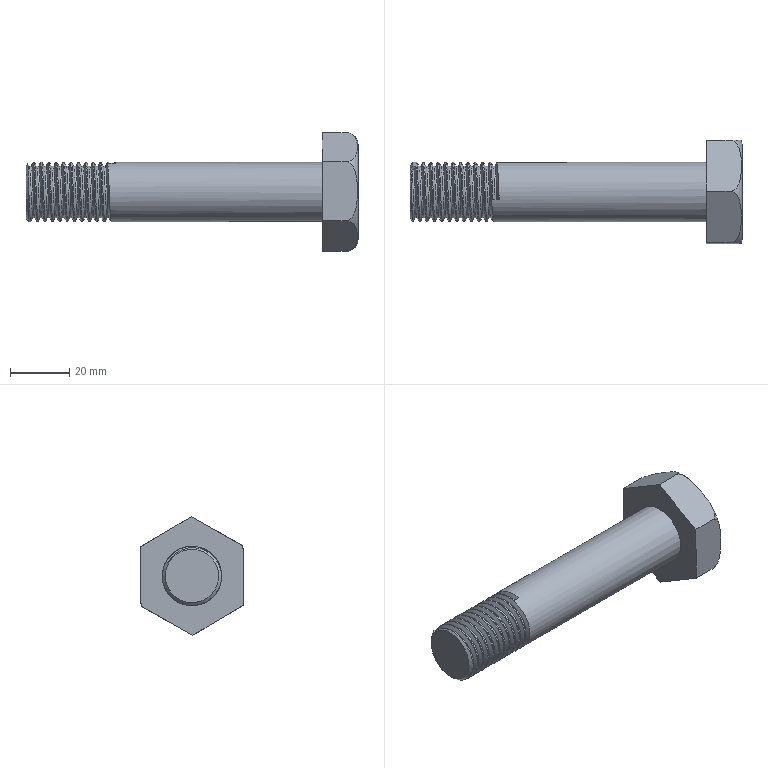Component | NX | CCJ-014 | 2 solids | 29 faces | volume 42449 mm3 | cylinder 13 | plane 12 | spline 2 | cone 1 | torus 1 | commonest cylinder face diameters 20 x12 17.5 x1